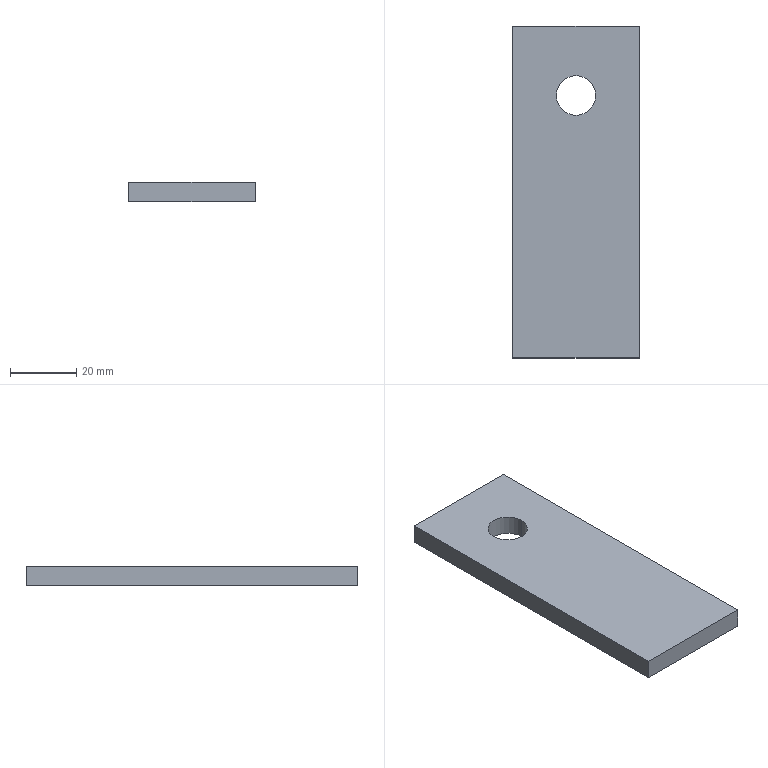Component | SolidWorks | HammerPiece-1_Blade-1 | 1 solid | 8 faces | box 38 x 100 x 6 mm | volume 22136 mm3 | plane 6 | cylinder 2 | commonest cylinder face diameters 11.872 x2
STEP:
#1=COLOUR_RGB('',0.7922,0.8196,0.9333);
#2=FILL_AREA_STYLE_COLOUR('',#1);
#3=FILL_AREA_STYLE('',(#2));
#4=SURFACE_STYLE_FILL_AREA(#3);
#5=SURFACE_SIDE_STYLE('',(#4));
#6=SURFACE_STYLE_USAGE(.BOTH.,#5);
#7=PRESENTATION_STYLE_ASSIGNMENT((#6));
#8=CARTESIAN_POINT('',(8.034,17.829,-4.449));
#9=VERTEX_POINT('',#8);
#10=CARTESIAN_POINT('',(8.501,17.829,-4.449));
#11=VERTEX_POINT('',#10);
#12=CARTESIAN_POINT('',(8.268,17.829,-4.449));
#13=DIRECTION('',(0.,0.,1.));
#14=DIRECTION('',(-1.,0.,0.));
#15=AXIS2_PLACEMENT_3D('',#12,#13,#14);
#16=CIRCLE('',#15,0.2337);
#17=EDGE_CURVE('',#9,#11,#16,.T.);
#18=ORIENTED_EDGE('',*,*,#17,.T.);
#19=CARTESIAN_POINT('',(8.501,17.829,-4.685));
#20=VERTEX_POINT('',#19);
#21=CARTESIAN_POINT('',(8.501,17.829,-4.449));
#22=DIRECTION('',(0.,0.,-1.));
#23=VECTOR('',#22,39.37);
#24=LINE('',#21,#23);
#25=EDGE_CURVE('',#11,#20,#24,.T.);
#26=ORIENTED_EDGE('',*,*,#25,.T.);
#27=CARTESIAN_POINT('',(8.034,17.829,-4.685));
#28=VERTEX_POINT('',#27);
#29=CARTESIAN_POINT('',(8.268,17.829,-4.685));
#30=DIRECTION('',(0.,0.,1.));
#31=DIRECTION('',(-1.,0.,0.));
#32=AXIS2_PLACEMENT_3D('',#29,#30,#31);
#33=CIRCLE('',#32,0.2337);
#34=EDGE_CURVE('',#28,#20,#33,.T.);
#35=ORIENTED_EDGE('',*,*,#34,.F.);
#36=CARTESIAN_POINT('',(8.034,17.829,-4.449));
#37=DIRECTION('',(0.,0.,-1.));
#38=VECTOR('',#37,39.37);
#39=LINE('',#36,#38);
#40=EDGE_CURVE('',#9,#28,#39,.T.);
#41=ORIENTED_EDGE('',*,*,#40,.F.);
#42=EDGE_LOOP('',(#18,#26,#35,#41));
#43=FACE_OUTER_BOUND('',#42,.T.);
#44=CARTESIAN_POINT('',(8.268,17.829,-4.449));
#45=DIRECTION('',(0.,0.,-1.));
#46=DIRECTION('',(-1.,0.,0.));
#47=AXIS2_PLACEMENT_3D('',#44,#45,#46);
#48=CYLINDRICAL_SURFACE('',#47,0.2337);
#49=ADVANCED_FACE('',(#43),#48,.F.);
#50=ORIENTED_EDGE('',*,*,#17,.F.);
#51=CARTESIAN_POINT('',(8.268,17.829,-4.449));
#52=DIRECTION('',(0.,0.,1.));
#53=DIRECTION('',(-1.,0.,0.));
#54=AXIS2_PLACEMENT_3D('',#51,#52,#53);
#55=CIRCLE('',#54,0.2337);
#56=EDGE_CURVE('',#11,#9,#55,.T.);
#57=ORIENTED_EDGE('',*,*,#56,.F.);
#58=EDGE_LOOP('',(#50,#57));
#59=FACE_BOUND('',#58,.T.);
#60=CARTESIAN_POINT('',(7.52,18.653,-4.449));
#61=VERTEX_POINT('',#60);
#62=CARTESIAN_POINT('',(9.016,18.653,-4.449));
#63=VERTEX_POINT('',#62);
#64=CARTESIAN_POINT('',(8.268,18.653,-4.449));
#65=DIRECTION('',(1.,0.,0.));
#66=VECTOR('',#65,39.37);
#67=LINE('',#64,#66);
#68=EDGE_CURVE('',#61,#63,#67,.T.);
#69=ORIENTED_EDGE('',*,*,#68,.F.);
#70=CARTESIAN_POINT('',(7.52,14.716,-4.449));
#71=VERTEX_POINT('',#70);
#72=CARTESIAN_POINT('',(7.52,8.839,-4.449));
#73=DIRECTION('',(0.,1.,0.));
#74=VECTOR('',#73,39.37);
#75=LINE('',#72,#74);
#76=EDGE_CURVE('',#71,#61,#75,.T.);
#77=ORIENTED_EDGE('',*,*,#76,.F.);
#78=CARTESIAN_POINT('',(9.016,14.716,-4.449));
#79=VERTEX_POINT('',#78);
#80=CARTESIAN_POINT('',(8.268,14.716,-4.449));
#81=DIRECTION('',(-1.,0.,0.));
#82=VECTOR('',#81,39.37);
#83=LINE('',#80,#82);
#84=EDGE_CURVE('',#79,#71,#83,.T.);
#85=ORIENTED_EDGE('',*,*,#84,.F.);
#86=CARTESIAN_POINT('',(9.016,8.839,-4.449));
#87=DIRECTION('',(0.,-1.,0.));
#88=VECTOR('',#87,39.37);
#89=LINE('',#86,#88);
#90=EDGE_CURVE('',#63,#79,#89,.T.);
#91=ORIENTED_EDGE('',*,*,#90,.F.);
#92=EDGE_LOOP('',(#69,#77,#85,#91));
#93=FACE_OUTER_BOUND('',#92,.T.);
#94=CARTESIAN_POINT('',(8.268,8.839,-4.449));
#95=DIRECTION('',(0.,0.,-1.));
#96=DIRECTION('',(-1.,0.,0.));
#97=AXIS2_PLACEMENT_3D('',#94,#95,#96);
#98=PLANE('',#97);
#99=ADVANCED_FACE('',(#59,#93),#98,.F.);
#100=ORIENTED_EDGE('',*,*,#25,.F.);
#101=ORIENTED_EDGE('',*,*,#56,.T.);
#102=ORIENTED_EDGE('',*,*,#40,.T.);
#103=CARTESIAN_POINT('',(8.268,17.829,-4.685));
#104=DIRECTION('',(0.,0.,1.));
#105=DIRECTION('',(-1.,0.,0.));
#106=AXIS2_PLACEMENT_3D('',#103,#104,#105);
#107=CIRCLE('',#106,0.2337);
#108=EDGE_CURVE('',#20,#28,#107,.T.);
#109=ORIENTED_EDGE('',*,*,#108,.F.);
#110=EDGE_LOOP('',(#100,#101,#102,#109));
#111=FACE_OUTER_BOUND('',#110,.T.);
#112=CARTESIAN_POINT('',(8.268,17.829,-4.449));
#113=DIRECTION('',(0.,0.,-1.));
#114=DIRECTION('',(-1.,0.,0.));
#115=AXIS2_PLACEMENT_3D('',#112,#113,#114);
#116=CYLINDRICAL_SURFACE('',#115,0.2337);
#117=ADVANCED_FACE('',(#111),#116,.F.);
#118=CARTESIAN_POINT('',(9.016,18.653,-4.685));
#119=VERTEX_POINT('',#118);
#120=CARTESIAN_POINT('',(9.016,18.653,-4.449));
#121=DIRECTION('',(0.,0.,-1.));
#122=VECTOR('',#121,39.37);
#123=LINE('',#120,#122);
#124=EDGE_CURVE('',#63,#119,#123,.T.);
#125=ORIENTED_EDGE('',*,*,#124,.F.);
#126=ORIENTED_EDGE('',*,*,#90,.T.);
#127=CARTESIAN_POINT('',(9.016,14.716,-4.685));
#128=VERTEX_POINT('',#127);
#129=CARTESIAN_POINT('',(9.016,14.716,-4.449));
#130=DIRECTION('',(0.,0.,1.));
#131=VECTOR('',#130,39.37);
#132=LINE('',#129,#131);
#133=EDGE_CURVE('',#128,#79,#132,.T.);
#134=ORIENTED_EDGE('',*,*,#133,.F.);
#135=CARTESIAN_POINT('',(9.016,18.653,-4.685));
#136=DIRECTION('',(-0.,-1.,0.));
#137=VECTOR('',#136,39.37);
#138=LINE('',#135,#137);
#139=EDGE_CURVE('',#119,#128,#138,.T.);
#140=ORIENTED_EDGE('',*,*,#139,.F.);
#141=EDGE_LOOP('',(#125,#126,#134,#140));
#142=FACE_OUTER_BOUND('',#141,.T.);
#143=CARTESIAN_POINT('',(9.016,18.653,-4.449));
#144=DIRECTION('',(-1.,0.,0.));
#145=DIRECTION('',(0.,1.,0.));
#146=AXIS2_PLACEMENT_3D('',#143,#144,#145);
#147=PLANE('',#146);
#148=ADVANCED_FACE('',(#142),#147,.F.);
#149=CARTESIAN_POINT('',(7.52,18.653,-4.685));
#150=VERTEX_POINT('',#149);
#151=CARTESIAN_POINT('',(7.52,18.653,-4.449));
#152=DIRECTION('',(0.,0.,-1.));
#153=VECTOR('',#152,39.37);
#154=LINE('',#151,#153);
#155=EDGE_CURVE('',#61,#150,#154,.T.);
#156=ORIENTED_EDGE('',*,*,#155,.F.);
#157=ORIENTED_EDGE('',*,*,#68,.T.);
#158=ORIENTED_EDGE('',*,*,#124,.T.);
#159=CARTESIAN_POINT('',(9.016,18.653,-4.685));
#160=DIRECTION('',(1.,0.,0.));
#161=VECTOR('',#160,39.37);
#162=LINE('',#159,#161);
#163=EDGE_CURVE('',#150,#119,#162,.T.);
#164=ORIENTED_EDGE('',*,*,#163,.F.);
#165=EDGE_LOOP('',(#156,#157,#158,#164));
#166=FACE_OUTER_BOUND('',#165,.T.);
#167=CARTESIAN_POINT('',(9.016,18.653,-4.449));
#168=DIRECTION('',(0.,-1.,0.));
#169=DIRECTION('',(-1.,0.,0.));
#170=AXIS2_PLACEMENT_3D('',#167,#168,#169);
#171=PLANE('',#170);
#172=ADVANCED_FACE('',(#166),#171,.F.);
#173=CARTESIAN_POINT('',(7.52,14.716,-4.685));
#174=VERTEX_POINT('',#173);
#175=CARTESIAN_POINT('',(7.52,14.716,-4.449));
#176=DIRECTION('',(0.,0.,-1.));
#177=VECTOR('',#176,39.37);
#178=LINE('',#175,#177);
#179=EDGE_CURVE('',#71,#174,#178,.T.);
#180=ORIENTED_EDGE('',*,*,#179,.F.);
#181=ORIENTED_EDGE('',*,*,#76,.T.);
#182=ORIENTED_EDGE('',*,*,#155,.T.);
#183=CARTESIAN_POINT('',(7.52,18.653,-4.685));
#184=DIRECTION('',(-0.,1.,0.));
#185=VECTOR('',#184,39.37);
#186=LINE('',#183,#185);
#187=EDGE_CURVE('',#174,#150,#186,.T.);
#188=ORIENTED_EDGE('',*,*,#187,.F.);
#189=EDGE_LOOP('',(#180,#181,#182,#188));
#190=FACE_OUTER_BOUND('',#189,.T.);
#191=CARTESIAN_POINT('',(7.52,18.653,-4.449));
#192=DIRECTION('',(1.,0.,0.));
#193=DIRECTION('',(0.,-1.,0.));
#194=AXIS2_PLACEMENT_3D('',#191,#192,#193);
#195=PLANE('',#194);
#196=ADVANCED_FACE('',(#190),#195,.F.);
#197=ORIENTED_EDGE('',*,*,#133,.T.);
#198=ORIENTED_EDGE('',*,*,#84,.T.);
#199=ORIENTED_EDGE('',*,*,#179,.T.);
#200=CARTESIAN_POINT('',(9.016,14.716,-4.685));
#201=DIRECTION('',(-1.,0.,0.));
#202=VECTOR('',#201,39.37);
#203=LINE('',#200,#202);
#204=EDGE_CURVE('',#128,#174,#203,.T.);
#205=ORIENTED_EDGE('',*,*,#204,.F.);
#206=EDGE_LOOP('',(#197,#198,#199,#205));
#207=FACE_OUTER_BOUND('',#206,.T.);
#208=CARTESIAN_POINT('',(9.016,14.716,-4.449));
#209=DIRECTION('',(0.,1.,0.));
#210=DIRECTION('',(1.,0.,0.));
#211=AXIS2_PLACEMENT_3D('',#208,#209,#210);
#212=PLANE('',#211);
#213=ADVANCED_FACE('',(#207),#212,.F.);
#214=ORIENTED_EDGE('',*,*,#34,.T.);
#215=ORIENTED_EDGE('',*,*,#108,.T.);
#216=EDGE_LOOP('',(#214,#215));
#217=FACE_BOUND('',#216,.T.);
#218=ORIENTED_EDGE('',*,*,#187,.T.);
#219=ORIENTED_EDGE('',*,*,#163,.T.);
#220=ORIENTED_EDGE('',*,*,#139,.T.);
#221=ORIENTED_EDGE('',*,*,#204,.T.);
#222=EDGE_LOOP('',(#218,#219,#220,#221));
#223=FACE_OUTER_BOUND('',#222,.T.);
#224=CARTESIAN_POINT('',(8.268,8.839,-4.685));
#225=DIRECTION('',(0.,0.,-1.));
#226=DIRECTION('',(-1.,0.,0.));
#227=AXIS2_PLACEMENT_3D('',#224,#225,#226);
#228=PLANE('',#227);
#229=ADVANCED_FACE('',(#217,#223),#228,.T.);
#230=CLOSED_SHELL('',(#49,#99,#117,#148,#172,#196,#213,#229));
#231=MANIFOLD_SOLID_BREP('',#230);
#232=STYLED_ITEM('',(#7),#231);
#233=(LENGTH_UNIT()NAMED_UNIT(*)SI_UNIT($,.METRE.));
#234=LENGTH_MEASURE_WITH_UNIT(LENGTH_MEASURE(0.0254),#233);
#235=DIMENSIONAL_EXPONENTS(1.,0.,0.,0.,0.,0.,0.);
#236=(CONVERSION_BASED_UNIT('',#234)LENGTH_UNIT()NAMED_UNIT(#235));
#237=UNCERTAINTY_MEASURE_WITH_UNIT(LENGTH_MEASURE(0.00001),#236,'','');
#238=(NAMED_UNIT(*)PLANE_ANGLE_UNIT()SI_UNIT($,.RADIAN.));
#239=(NAMED_UNIT(*)SI_UNIT($,.STERADIAN.)SOLID_ANGLE_UNIT());
#240=(GEOMETRIC_REPRESENTATION_CONTEXT(3)GLOBAL_UNCERTAINTY_ASSIGNED_CONTEXT((#237))GLOBAL_UNIT_ASSIGNED_CONTEXT((#236,#238,#239))REPRESENTATION_CONTEXT('',''));
#241=MECHANICAL_DESIGN_GEOMETRIC_PRESENTATION_REPRESENTATION('',(#232),#240);
#242=PRESENTATION_LAYER_ASSIGNMENT('','',(#232));
#243=CARTESIAN_POINT('',(0.,0.,0.));
#244=DIRECTION('',(0.,0.,1.));
#245=DIRECTION('',(1.,0.,0.));
#246=AXIS2_PLACEMENT_3D('',#243,#244,#245);
#247=(LENGTH_UNIT()NAMED_UNIT(*)SI_UNIT($,.METRE.));
#248=LENGTH_MEASURE_WITH_UNIT(LENGTH_MEASURE(0.0254),#247);
#249=DIMENSIONAL_EXPONENTS(1.,0.,0.,0.,0.,0.,0.);
#250=(CONVERSION_BASED_UNIT('',#248)LENGTH_UNIT()NAMED_UNIT(#249));
#251=UNCERTAINTY_MEASURE_WITH_UNIT(LENGTH_MEASURE(0.00001),#250,'','');
#252=(NAMED_UNIT(*)PLANE_ANGLE_UNIT()SI_UNIT($,.RADIAN.));
#253=(NAMED_UNIT(*)SI_UNIT($,.STERADIAN.)SOLID_ANGLE_UNIT());
#254=(GEOMETRIC_REPRESENTATION_CONTEXT(3)GLOBAL_UNCERTAINTY_ASSIGNED_CONTEXT((#251))GLOBAL_UNIT_ASSIGNED_CONTEXT((#250,#252,#253))REPRESENTATION_CONTEXT('',''));
#255=ADVANCED_BREP_SHAPE_REPRESENTATION('',(#231,#246),#254);